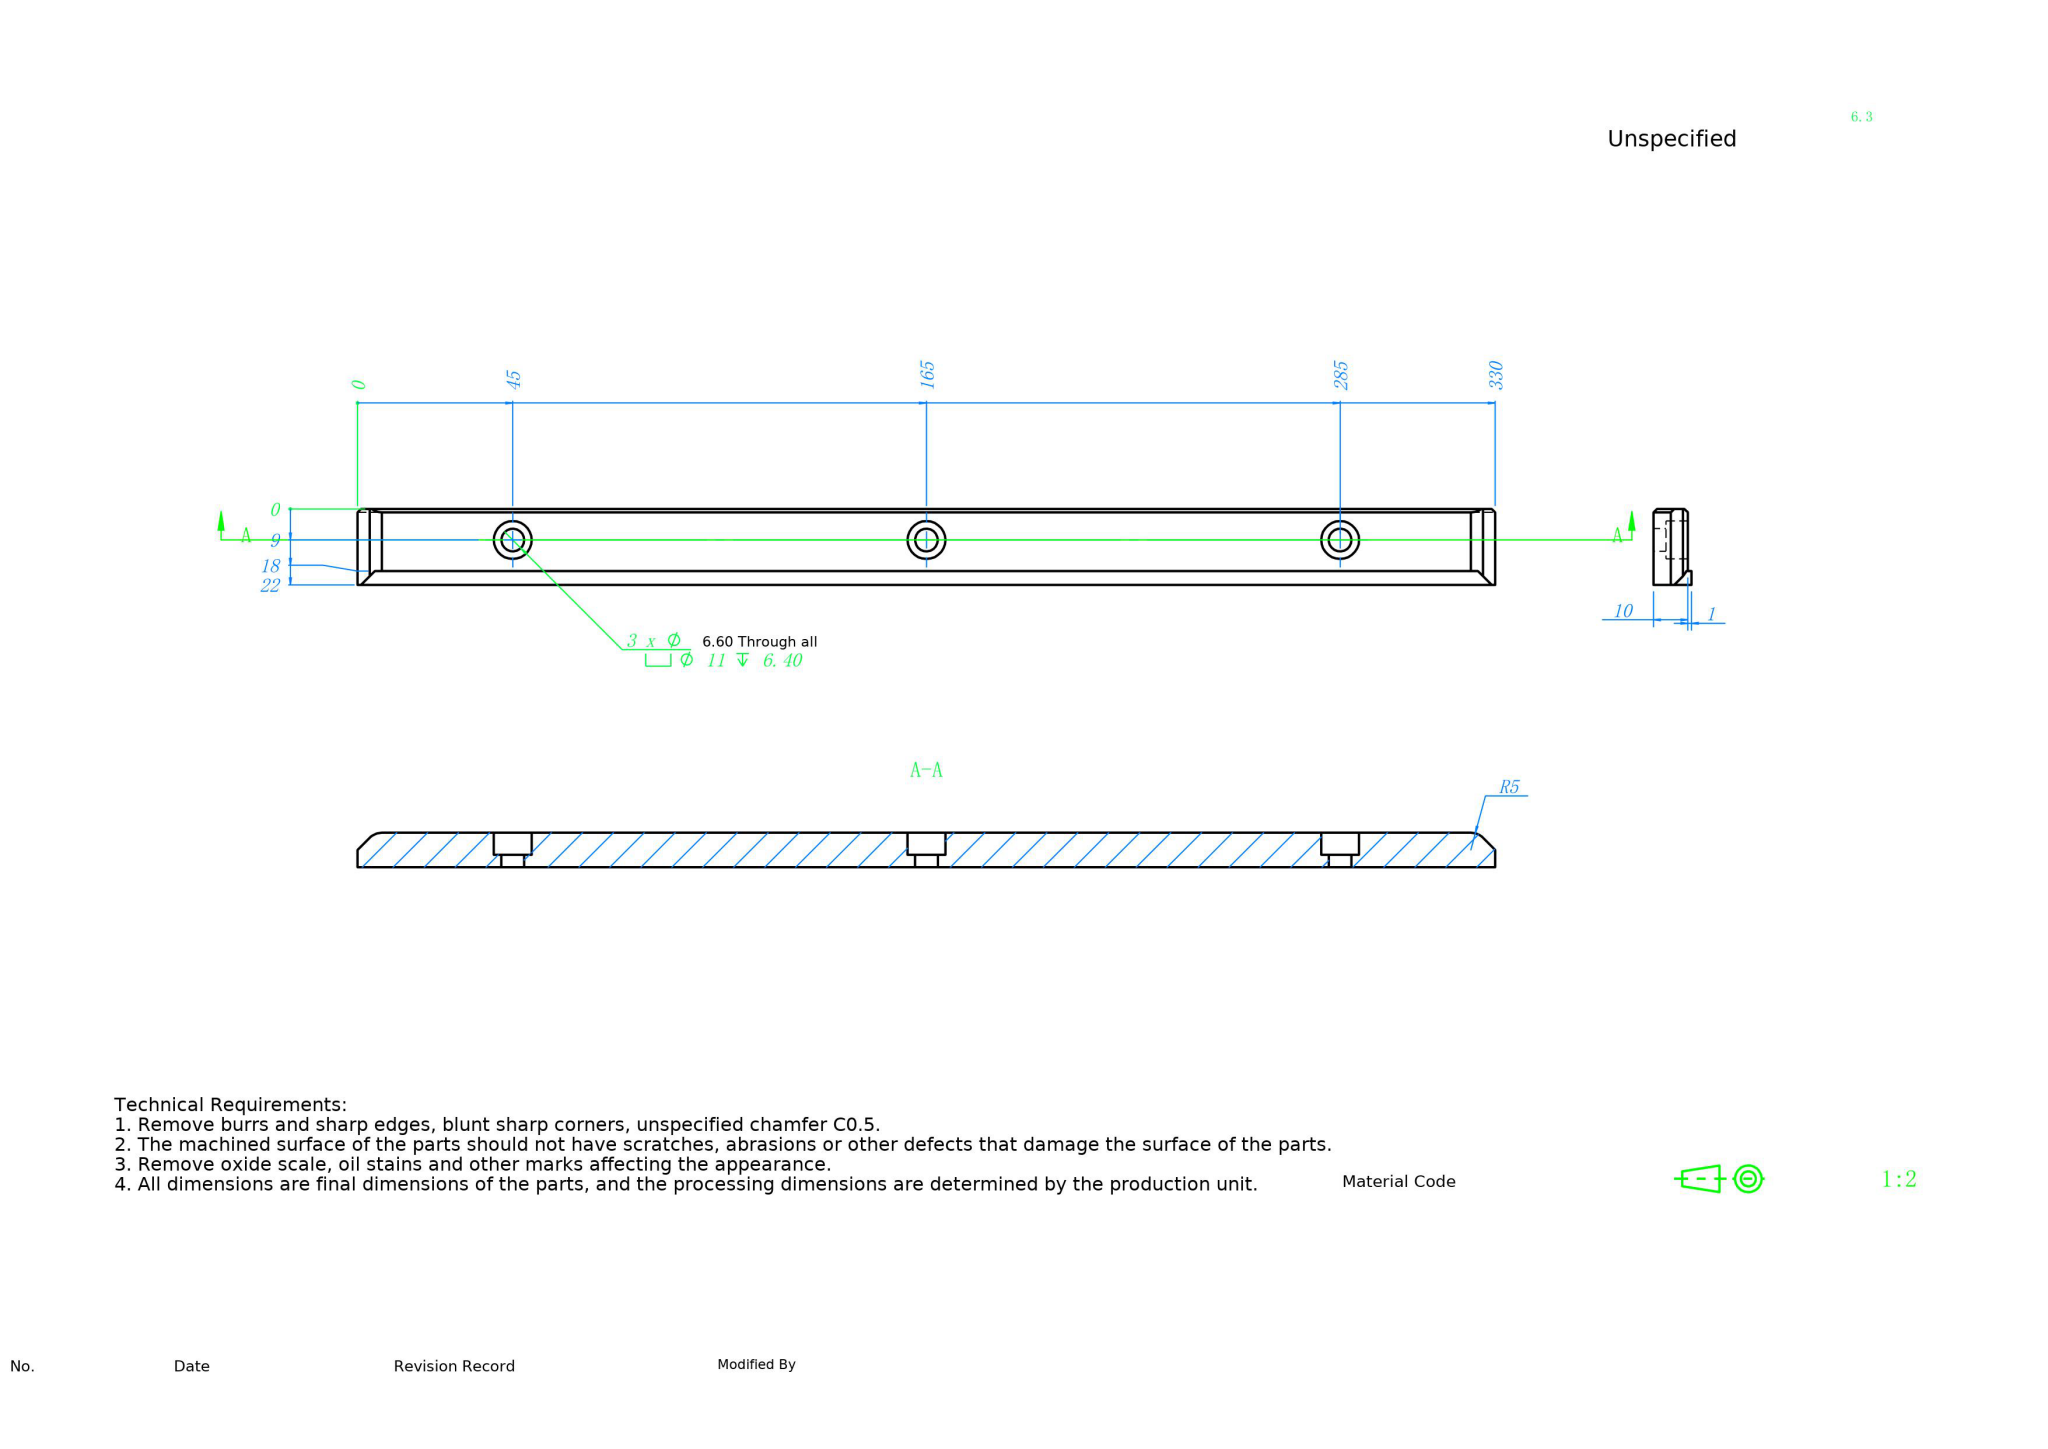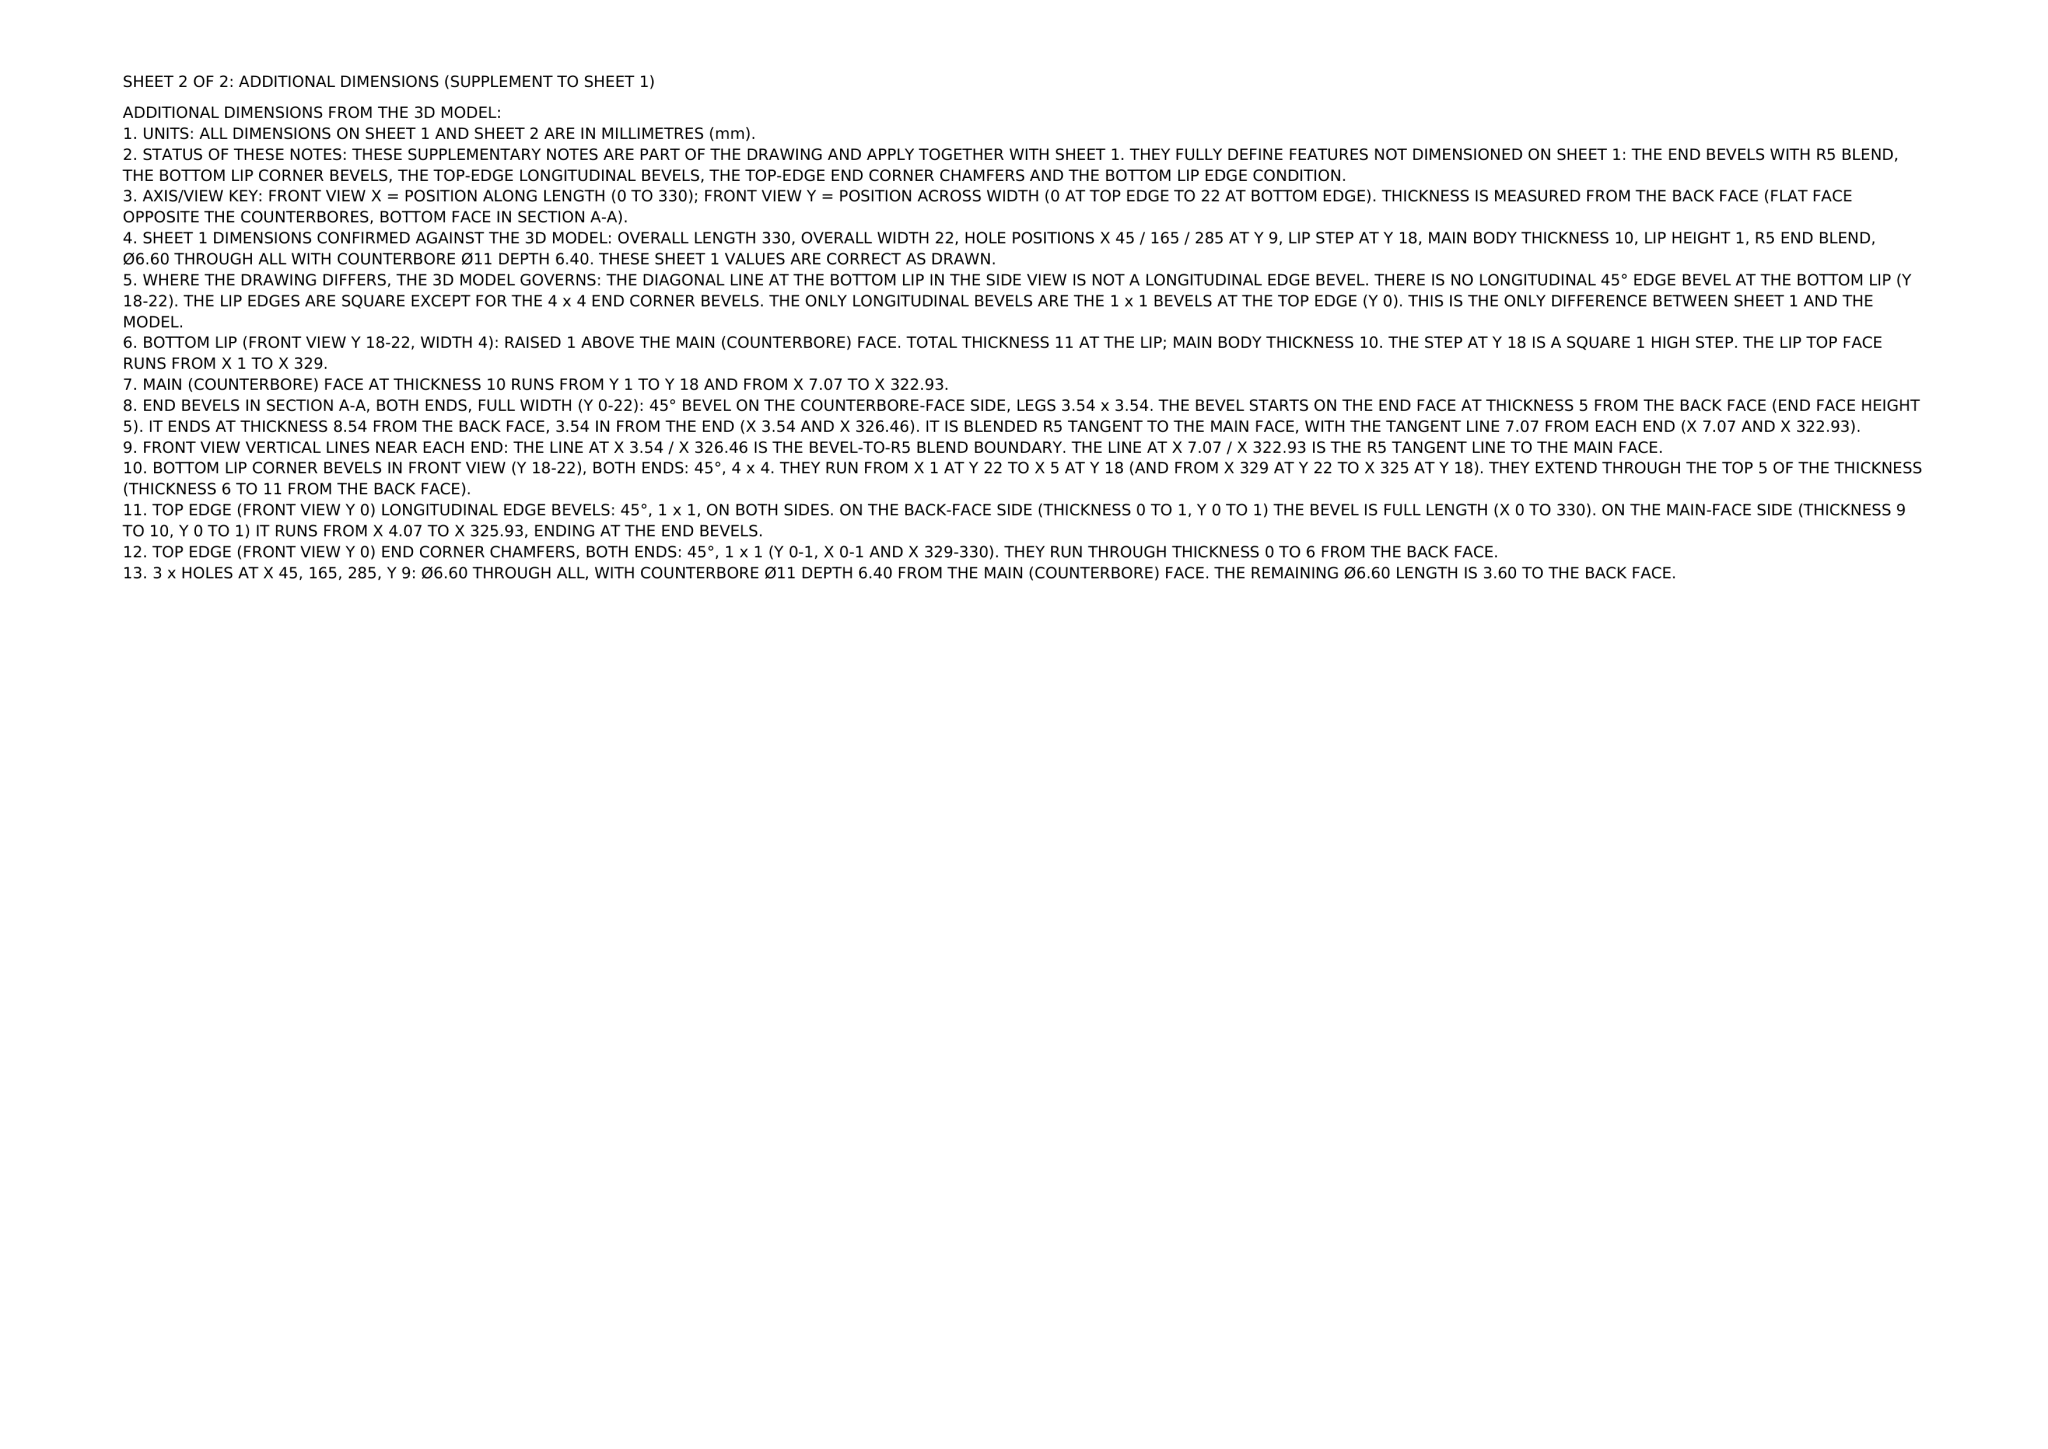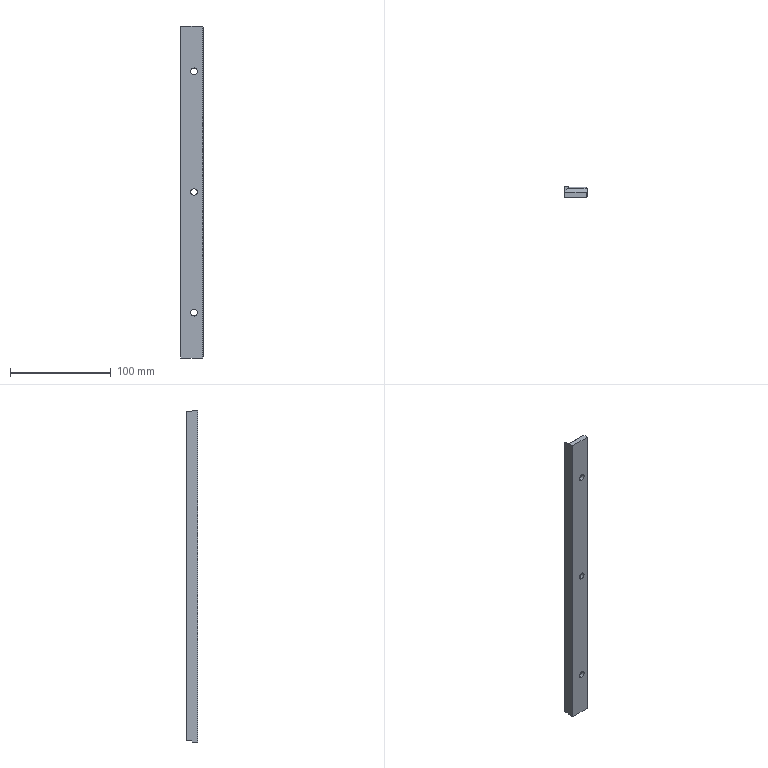Part | NX | mm | 1 solid | 33 faces | box 22 x 11 x 330 mm | volume 70824 mm3 | plane 19 | cylinder 14 | commonest cylinder face diameters 11 x6 6.6 x6 10 x2